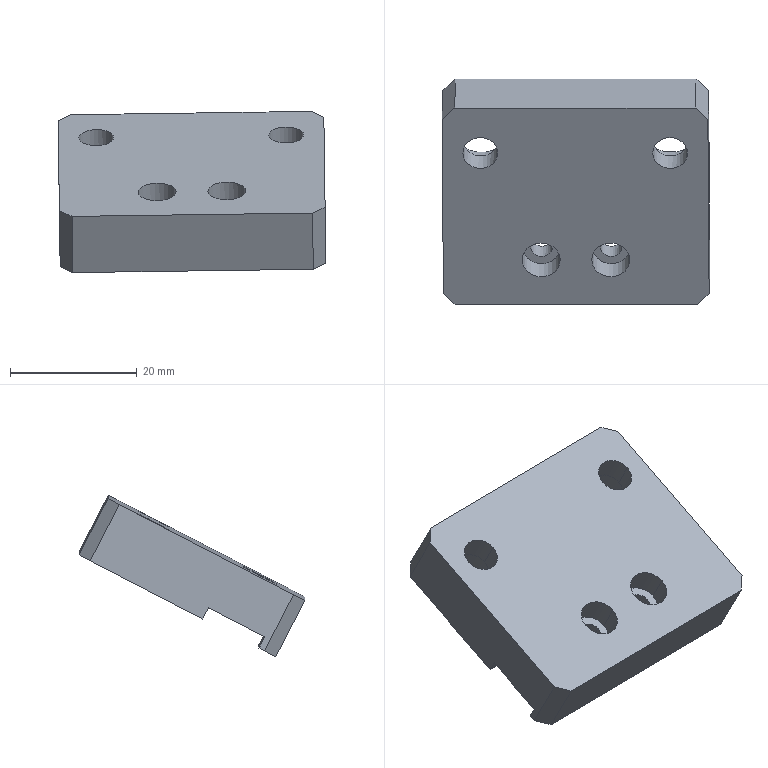Component | SolidWorks | 2018SOLIDWORKS1400000016-1 | 1 solid | 34 faces | box 42.32 x 35.69 x 25.47 mm | volume 12362 mm3 | plane 18 | cylinder 16 | commonest cylinder face diameters 6 x4 3.4 x4 10 x4 5.5 x4 | material 6061 Alloy
build123d program:
from build123d import *

# Parameters (mm, degrees)
SKETCH1_W                                          = 42
SKETCH1_H                                          = 35
BOSS_EXTRUDE1_DEPTH                                = 5
SKETCH2_W                                          = 42
SKETCH2_H                                          = 10
CUT_EXTRUDE1_DEPTH                                 = 2
HOLE_SIZE_ACCORDING_TO_TYPE_1_OF_HEXAG_D           = 5.5
HOLE_SIZE_ACCORDING_TO_TYPE_1_OF_HEXAG_CBORE_D     = 10
HOLE_SIZE_ACCORDING_TO_TYPE_1_OF_HEXAG_CBORE_DEPTH = 5.7
CHAMFER1_SIZE                                      = 2
HOLE_SIZE_ACCORDING_TO_TYPE_2_OF_HEXAG_D           = 3.4
HOLE_SIZE_ACCORDING_TO_TYPE_2_OF_HEXAG_CBORE_D     = 6
HOLE_SIZE_ACCORDING_TO_TYPE_2_OF_HEXAG_CBORE_DEPTH = 4.5


with BuildPart() as part:
    # Sketch1 → Boss-Extrude1 (new, symmetric)
    with BuildSketch(Plane.XY):
        Rectangle(SKETCH1_W, SKETCH1_H)
    extrude(amount=BOSS_EXTRUDE1_DEPTH, both=True)

    # Sketch2 → Cut-Extrude1 (cut)
    with BuildSketch(Plane(origin=(0, 0, -5), x_dir=(-1, 0, 0), z_dir=(0, 0, -1))):
        with Locations((0, 9.5)):
            Rectangle(SKETCH2_W, SKETCH2_H)
    extrude(amount=-CUT_EXTRUDE1_DEPTH, mode=Mode.SUBTRACT)

    # Hole Size _according to_ Type 1 of Hexag (through all)
    with Locations(Plane(origin=(0, 0, -5), x_dir=(-1, 0, 0), z_dir=(0, 0, -1))):
        with Locations((-15, -9.5), (15, -9.5)):
            CounterBoreHole(HOLE_SIZE_ACCORDING_TO_TYPE_1_OF_HEXAG_D / 2, HOLE_SIZE_ACCORDING_TO_TYPE_1_OF_HEXAG_CBORE_D / 2, HOLE_SIZE_ACCORDING_TO_TYPE_1_OF_HEXAG_CBORE_DEPTH)

    # Chamfer1
    chamfer1_edges = [part.edges().sort_by_distance(p)[0] for p in [
        (21, -17.5, 0),
        (-21, -17.5, 0),
        (-21, 17.5, 0),
        (21, 17.5, 0),
    ]]
    chamfer(chamfer1_edges, length=CHAMFER1_SIZE)

    # Hole Size _according to_ Type 2 of Hexag (through all)
    with Locations(Plane.XY.offset(5)):
        with Locations((5.5, 9.5), (-5.5, 9.5)):
            CounterBoreHole(HOLE_SIZE_ACCORDING_TO_TYPE_2_OF_HEXAG_D / 2, HOLE_SIZE_ACCORDING_TO_TYPE_2_OF_HEXAG_CBORE_D / 2, HOLE_SIZE_ACCORDING_TO_TYPE_2_OF_HEXAG_CBORE_DEPTH)


solid = part.part

# Placed as in the assembly
solid = solid.moved(Location((96.907, -39.508, 162.818), (27.325, -0.7042, -179.636)))